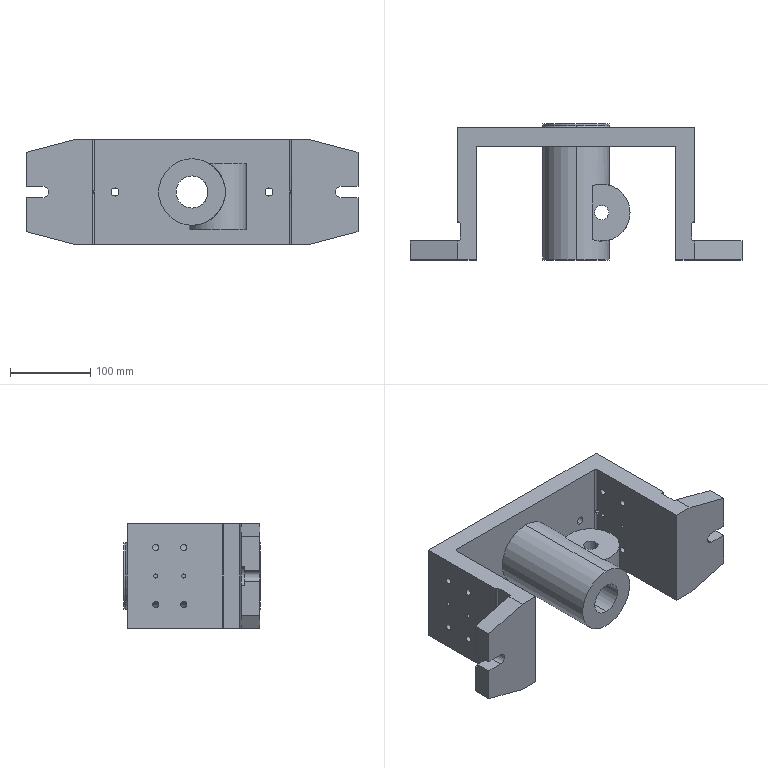Component | SolidWorks | DrillJigBody-1 | 1 solid | 115 faces | box 414.01 x 169.66 x 130 mm | volume 2706781 mm3 | cylinder 62 | plane 39 | cone 12 | torus 2 | commonest cylinder face diameters 8 x16 10 x8 5 x8 4 x6 4.732 x6 83 x4 44 x2 17.836 x2
build123d program:
from build123d import *

# Parameters (mm, degrees)
BOSS_EXTRUDE1_DEPTH                 = 65
CUT_EXTRUDE1_DEPTH                  = 118
CUT_EXTRUDE2_DEPTH                  = 118
CUT_EXTRUDE3_DEPTH                  = 4
SKETCH5_R                           = 41.5
BOSS_EXTRUDE2_DEPTH                 = 4
FILLET1_R                           = 2
BOSS_EXTRUDE3_START                 = 142
SKETCH7_R                           = 41.5
BOSS_EXTRUDE3_DEPTH                 = 142
SKETCH9_R                           = 35.5
BOSS_EXTRUDE4_DEPTH                 = 83
SKETCH11_R                          = 20
CUT_EXTRUDE5_DEPTH                  = 193
CIRPATTERN1_COUNT                   = 3
M10_TAPPED_HOLE1_AT_2_COUNT         = 2
M10_TAPPED_HOLE1_AT_2_PITCH         = 32
M8_TAPPED_HOLE1_AT_2_COUNT          = 2
M8_TAPPED_HOLE1_AT_2_PITCH          = 71
M8_TAPPED_HOLE1_AT_3_COUNT          = 2
M8_TAPPED_HOLE1_AT_3_PITCH          = 79.158
M8_TAPPED_HOLE1_AT_4_COUNT          = 2
M8_TAPPED_HOLE1_AT_4_PITCH          = 35
SIZE_MM_DOWEL_PIN_HOLE_1_AT_2_COUNT = 2
SIZE_MM_DOWEL_PIN_HOLE_1_AT_2_PITCH = 35
SPLIT1_SURFACE_1_BACK               = 466.931
SPLIT1_SURFACE_1_DEPTH              = 933.862
SPLIT1_SURFACE_2_BACK               = 466.931
SPLIT1_SURFACE_2_DEPTH              = 933.862


with BuildPart() as part:
    # Model → Boss-Extrude1 (new, symmetric)
    with BuildSketch(Plane.XY):
        with BuildLine():
            Line((-207.007, 0), (-207.007, 23.658))
            Line((-207.007, 23.658), (-147.862, 23.658))
            Line((-147.862, 23.658), (-146.679, 23.658))
            ThreePointArc((-146.679, 23.658), (-145.006, 24.351), (-144.313, 26.024))
            Line((-144.313, 26.024), (-144.313, 44.95))
            ThreePointArc((-144.313, 44.95), (-145.006, 46.623), (-146.679, 47.316))
            Line((-146.679, 47.316), (-147.862, 47.316))
            Line((-147.862, 47.316), (-147.862, 165.606))
            Line((-147.862, 165.606), (147.862, 165.606))
            Line((147.862, 165.606), (147.862, 47.316))
            Line((147.862, 47.316), (146.679, 47.316))
            ThreePointArc((146.679, 47.316), (145.006, 46.623), (144.313, 44.95))
            Line((144.313, 44.95), (144.313, 26.024))
            ThreePointArc((144.313, 26.024), (145.006, 24.351), (146.679, 23.658))
            Line((146.679, 23.658), (147.862, 23.658))
            Line((147.862, 23.658), (207.007, 23.658))
            Line((207.007, 23.658), (207.007, 0))
            Line((207.007, 0), (147.862, 0))
            Line((147.862, 0), (124.204, 0))
            Line((124.204, 0), (124.204, 139.582))
            ThreePointArc((124.204, 139.582), (123.511, 141.255), (121.838, 141.948))
            Line((121.838, 141.948), (42.805, 141.948))
            Line((42.805, 141.948), (-42.805, 141.948))
            Line((-42.805, 141.948), (-121.838, 141.948))
            ThreePointArc((-121.838, 141.948), (-123.511, 141.255), (-124.204, 139.582))
            Line((-124.204, 139.582), (-124.204, 0))
            Line((-124.204, 0), (-147.862, 0))
            Line((-147.862, 0), (-207.007, 0))
        make_face()
    extrude(amount=BOSS_EXTRUDE1_DEPTH, both=True)

    # Sketch2 → Cut-Extrude1 (cut)
    with BuildSketch(Plane(origin=(0, 23.658, 0), x_dir=(1, 0, 0), z_dir=(0, 1, 0))):
        Polygon((-207.007, 49.5), (-147.862, 65), (-207.007, 65), align=None)
        Polygon((-207.007, -65), (-147.862, -65), (-207.007, -49.5), align=None)
    cut_extrude1 = extrude(amount=-CUT_EXTRUDE1_DEPTH, mode=Mode.SUBTRACT)

    # Mirror1: Cut-Extrude1 across plane
    add(cut_extrude1.mirror(Plane(origin=(0, 0, 0), x_dir=(0, 0, 1), z_dir=(1, 0, 0))), mode=Mode.SUBTRACT)

    # Sketch3 → Cut-Extrude2 (cut)
    with BuildSketch(Plane(origin=(0, 23.658, 0), x_dir=(1, 0, 0), z_dir=(0, 1, 0))):
        with BuildLine():
            Line((-186.007, 7), (-207.007, 7))
            Line((-207.007, 7), (-207.007, -7))
            Line((-207.007, -7), (-186.007, -7))
            ThreePointArc((-186.007, -7), (-179.007, 0), (-186.007, 7))
        make_face()
    cut_extrude2 = extrude(amount=-CUT_EXTRUDE2_DEPTH, mode=Mode.SUBTRACT)

    # Sketch4 → Cut-Extrude3 (cut)
    with BuildSketch(Plane(origin=(0, 23.658, 0), x_dir=(1, 0, 0), z_dir=(0, 1, 0))):
        with BuildLine():
            Line((-186.007, 12), (-207.007, 12))
            Line((-207.007, 12), (-207.007, 7))
            Line((-207.007, 7), (-186.007, 7))
            ThreePointArc((-186.007, 7), (-179.007, 0), (-186.007, -7))
            Line((-186.007, -7), (-207.007, -7))
            Line((-207.007, -7), (-207.007, -12))
            Line((-207.007, -12), (-186.007, -12))
            ThreePointArc((-186.007, -12), (-174.007, 0), (-186.007, 12))
        make_face()
    cut_extrude3 = extrude(amount=-CUT_EXTRUDE3_DEPTH, mode=Mode.SUBTRACT)

    # Mirror2: Cut-Extrude2, Cut-Extrude3 across plane
    add(cut_extrude2.mirror(Plane(origin=(0, 0, 0), x_dir=(0, 0, 1), z_dir=(1, 0, 0))), mode=Mode.SUBTRACT)
    add(cut_extrude3.mirror(Plane(origin=(0, 0, 0), x_dir=(0, 0, 1), z_dir=(1, 0, 0))), mode=Mode.SUBTRACT)

    # Sketch5 → Boss-Extrude2 (add)
    with BuildSketch(Plane(origin=(0, 165.606, 0), x_dir=(1, 0, 0), z_dir=(0, 1, 0))):
        with Locations(Location((0, 0, 0), (0, 0, 270))):
            Circle(SKETCH5_R)
    extrude(amount=BOSS_EXTRUDE2_DEPTH)

    # Fillet1
    fillet1_edges = [part.edges().sort_by_distance(p)[0] for p in [
        (0, 165.606, -41.5),
    ]]
    fillet(fillet1_edges, radius=FILLET1_R)

    # Sketch7 → Boss-Extrude3 (add)
    with BuildSketch(Plane.XZ.offset(-141.948).offset(BOSS_EXTRUDE3_START)):
        with Locations(Location((0, 0, 0), (0, 0, 270))):
            Circle(SKETCH7_R)
    extrude(amount=-BOSS_EXTRUDE3_DEPTH)

    # Sketch9 → Boss-Extrude4 (add)
    with BuildSketch(Plane.XY.offset(47)):
        with Locations((32, 58.948)):
            Circle(SKETCH9_R)
    extrude(amount=-BOSS_EXTRUDE4_DEPTH)

    # Sketch10 → Cut-Revolve1 (revolve, cut)
    with BuildSketch(Plane(origin=(0, 58.948, 0), x_dir=(-1, 0, 0), z_dir=(0, -1, 0))):
        Polygon((-32, -47), (-54, -47), (-54, -43), (-49.918, -22), (-49.918, 19), (-40.918, 19), (-40.918, 36), (-32, 36), align=None)
    revolve(axis=Axis((32, 58.948, 81.865), (0, 0, -1)), mode=Mode.SUBTRACT)

    # Sketch11 → Cut-Extrude5 (cut)
    with BuildSketch(Plane(origin=(0, 169.606, 0), x_dir=(1, 0, 0), z_dir=(0, 1, 0))):
        with Locations(Location((0, 0, 0), (0, 0, 270))):
            Circle(SKETCH11_R)
    extrude(amount=-CUT_EXTRUDE5_DEPTH, mode=Mode.SUBTRACT)

    # Sketch13 → M4 Tapped Hole1 (revolve, cut)
    with BuildSketch(Plane(origin=(32, 29.448, 47), x_dir=(0, -1, 0), z_dir=(1, 0, 0))):
        Polygon((0, 0), (0, 16.702), (2, 15.5), (2, 0), align=None)
    m4_tapped_hole1 = revolve(axis=Axis((32, 29.448, 53.35), (0, 0, -1)), mode=Mode.SUBTRACT)

    # CirPattern1: M4 Tapped Hole1 ×3 about axis
    cirpattern1_axis = Axis((32, 58.948, 0), (0, 0, 1))
    for i in range(1, CIRPATTERN1_COUNT):
        add(m4_tapped_hole1.rotate(cirpattern1_axis, i * 360 / CIRPATTERN1_COUNT), mode=Mode.SUBTRACT)

    # Sketch15 → M10 Tapped Hole1 (revolve, cut)
    with BuildSketch(Plane(origin=(-96, 165.606, 0), x_dir=(0, 0, 1), z_dir=(1, 0, 0))):
        Polygon((0, 0), (0, 31.004), (5, 28), (5, 0), align=None)
    m10_tapped_hole1 = revolve(axis=Axis((-96, 171.956, 0), (0, -1, 0)), mode=Mode.SUBTRACT)

    # M10 Tapped Hole1 at 2: M10 Tapped Hole1 ×2
    with Locations(*[(-i * M10_TAPPED_HOLE1_AT_2_PITCH, 0, 0) for i in range(1, M10_TAPPED_HOLE1_AT_2_COUNT)]):
        add(m10_tapped_hole1, mode=Mode.SUBTRACT)

    # Mirror3: M10 Tapped Hole1 across plane
    add(m10_tapped_hole1.mirror(Plane(origin=(0, 0, 0), x_dir=(0, 0, 1), z_dir=(1, 0, 0))), mode=Mode.SUBTRACT)

    # Mirror3 copy 1 sketch → Mirror3 copy 1 (revolve, cut)
    with BuildSketch(Plane(origin=(128, 165.606, 0), x_dir=(0, 0, 1), z_dir=(-1, 0, 0))):
        Polygon((0, 0), (0, -31.004), (5, -28), (5, 0), align=None)
    revolve(axis=Axis((128, 171.956, 0), (0, 1, 0)), mode=Mode.SUBTRACT)

    # Sketch17 → M8 Tapped Hole1 (revolve, cut)
    with BuildSketch(Plane(origin=(-147.862, 130, -35.5), x_dir=(0, 0, 1), z_dir=(0, 1, 0))):
        Polygon((0, 0), (0, 38.653), (4, 36.25), (4, 0), align=None)
    m8_tapped_hole1 = revolve(axis=Axis((-154.212, 130, -35.5), (1, 0, 0)), mode=Mode.SUBTRACT)

    # M8 Tapped Hole1 at 2: M8 Tapped Hole1 ×2
    with Locations(*[(0, 0, i * M8_TAPPED_HOLE1_AT_2_PITCH) for i in range(1, M8_TAPPED_HOLE1_AT_2_COUNT)]):
        add(m8_tapped_hole1, mode=Mode.SUBTRACT)

    # M8 Tapped Hole1 at 3: M8 Tapped Hole1 ×2
    with Locations(*[Vector(0, -0.4422, 0.8969) * (i * M8_TAPPED_HOLE1_AT_3_PITCH) for i in range(1, M8_TAPPED_HOLE1_AT_3_COUNT)]):
        add(m8_tapped_hole1, mode=Mode.SUBTRACT)

    # M8 Tapped Hole1 at 4: M8 Tapped Hole1 ×2
    with Locations(*[(0, -i * M8_TAPPED_HOLE1_AT_4_PITCH, 0) for i in range(1, M8_TAPPED_HOLE1_AT_4_COUNT)]):
        add(m8_tapped_hole1, mode=Mode.SUBTRACT)

    # Sketch19 → Size mm Dowel Pin Hole 1 (revolve, cut)
    with BuildSketch(Plane(origin=(-147.862, 130, 0), x_dir=(0, 0, 1), z_dir=(0, 1, 0))):
        Polygon((0, 0), (0, 37.752), (2.5, 36.25), (2.5, 0), align=None)
    size_mm_dowel_pin_hole_1 = revolve(axis=Axis((-154.212, 130, 0), (1, 0, 0)), mode=Mode.SUBTRACT)

    # Size mm Dowel Pin Hole 1 at 2: Size mm Dowel Pin Hole 1 ×2
    with Locations(*[(0, -i * SIZE_MM_DOWEL_PIN_HOLE_1_AT_2_PITCH, 0) for i in range(1, SIZE_MM_DOWEL_PIN_HOLE_1_AT_2_COUNT)]):
        add(size_mm_dowel_pin_hole_1, mode=Mode.SUBTRACT)

    # Mirror4: M8 Tapped Hole1, Size mm Dowel Pin Hole 1 across plane
    add(m8_tapped_hole1.mirror(Plane(origin=(0, 0, 0), x_dir=(0, 0, 1), z_dir=(1, 0, 0))), mode=Mode.SUBTRACT)
    add(size_mm_dowel_pin_hole_1.mirror(Plane(origin=(0, 0, 0), x_dir=(0, 0, 1), z_dir=(1, 0, 0))), mode=Mode.SUBTRACT)

    # Mirror4 copy 1 sketch → Mirror4 copy 1 (revolve, cut)
    with BuildSketch(Plane(origin=(147.862, 130, 35.5), x_dir=(0, 0, 1), z_dir=(0, 1, 0))):
        Polygon((0, 0), (0, -38.653), (4, -36.25), (4, 0), align=None)
    revolve(axis=Axis((154.212, 130, 35.5), (1, 0, 0)), mode=Mode.SUBTRACT)

    # Mirror4 copy 2 sketch → Mirror4 copy 2 (revolve, cut)
    with BuildSketch(Plane(origin=(147.862, 95, 35.5), x_dir=(0, 0, 1), z_dir=(0, 1, 0))):
        Polygon((0, 0), (0, -38.653), (4, -36.25), (4, 0), align=None)
    revolve(axis=Axis((154.212, 95, 35.5), (1, 0, 0)), mode=Mode.SUBTRACT)

    # Mirror4 copy 3 sketch → Mirror4 copy 3 (revolve, cut)
    with BuildSketch(Plane(origin=(147.862, 95, -35.5), x_dir=(0, 0, 1), z_dir=(0, 1, 0))):
        Polygon((0, 0), (0, -38.653), (4, -36.25), (4, 0), align=None)
    revolve(axis=Axis((154.212, 95, -35.5), (1, 0, 0)), mode=Mode.SUBTRACT)

    # Mirror4 copy 4 sketch → Mirror4 copy 4 (revolve, cut)
    with BuildSketch(Plane(origin=(147.862, 95, 0), x_dir=(0, 0, 1), z_dir=(0, 1, 0))):
        Polygon((0, 0), (0, -37.752), (2.5, -36.25), (2.5, 0), align=None)
    revolve(axis=Axis((154.212, 95, 0), (1, 0, 0)), mode=Mode.SUBTRACT)


with BuildPart() as body_2:
    # Split1: the piece behind the surface
    add(part.part)
    # Split1 surface: a surface, the sketch's curves swept straight by 933.862 mm
    with BuildLine(Plane(origin=(0, 0, -65), x_dir=(-1, 0, 0), z_dir=(0, 0, -1)).offset(-SPLIT1_SURFACE_1_BACK), mode=Mode.PRIVATE) as split1_surface_1_path:
        Line((-102.385, 141.948), (63.991, 141.948))
        Line((63.991, 141.948), (63.991, -61.217))
        Line((63.991, -61.217), (-102.385, -61.217))
        Line((-102.385, -61.217), (-102.385, 141.948))
    split1_surface_1 = Shell.extrude(split1_surface_1_path.wire(), (0 * SPLIT1_SURFACE_1_DEPTH, 0 * SPLIT1_SURFACE_1_DEPTH, -1 * SPLIT1_SURFACE_1_DEPTH))
    split(bisect_by=split1_surface_1, keep=Keep.BOTTOM)


with BuildPart() as part_1:
    add(part.part)

    # Split1: split by a surface, the side it looks to stays
    # Split1 surface: a surface, the sketch's curves swept straight by 933.862 mm
    with BuildLine(Plane(origin=(0, 0, -65), x_dir=(-1, 0, 0), z_dir=(0, 0, -1)).offset(-SPLIT1_SURFACE_2_BACK), mode=Mode.PRIVATE) as split1_surface_2_path:
        Line((-102.385, 141.948), (63.991, 141.948))
        Line((63.991, 141.948), (63.991, -61.217))
        Line((63.991, -61.217), (-102.385, -61.217))
        Line((-102.385, -61.217), (-102.385, 141.948))
    split1_surface_2 = Shell.extrude(split1_surface_2_path.wire(), (0 * SPLIT1_SURFACE_2_DEPTH, 0 * SPLIT1_SURFACE_2_DEPTH, -1 * SPLIT1_SURFACE_2_DEPTH))
    split(bisect_by=split1_surface_2, keep=Keep.TOP)


with BuildPart() as body_3:
    # Mirror5: mirrored copy
    add(body_2.part.mirror(Plane(origin=(0, 0, 0), x_dir=(1, 0, 0), z_dir=(0, 0, -1))))


with BuildPart() as part_2:
    add(part_1.part)

    # Combine1: union body 3
    add(body_3.part)


solid = part_2.part